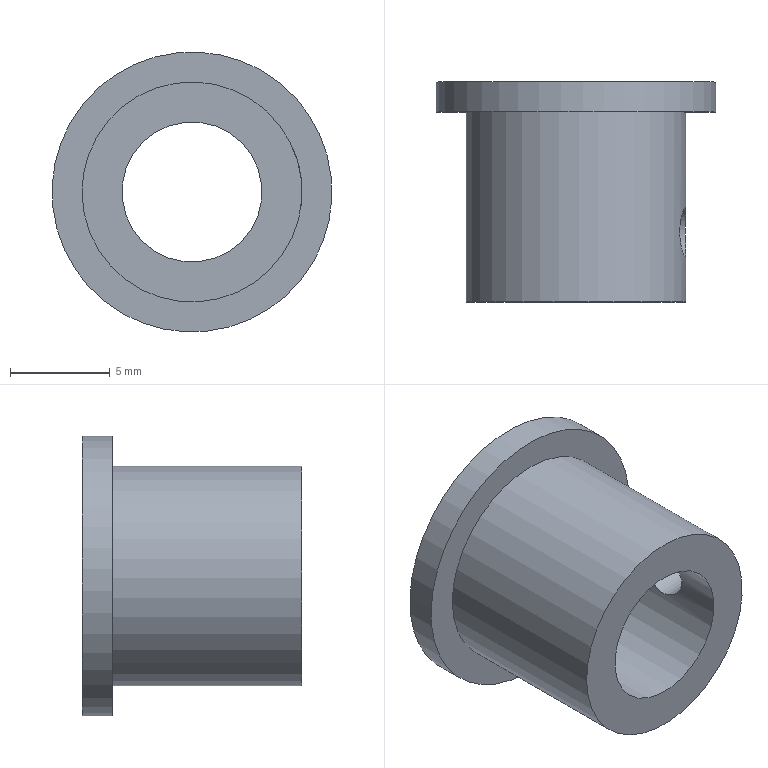Component | NX | BEARING | 1 solid | 7 faces | volume 700 mm3 | cylinder 4 | plane 3 | commonest cylinder face diameters 11 x1 7 x1 14 x1 2.5 x1